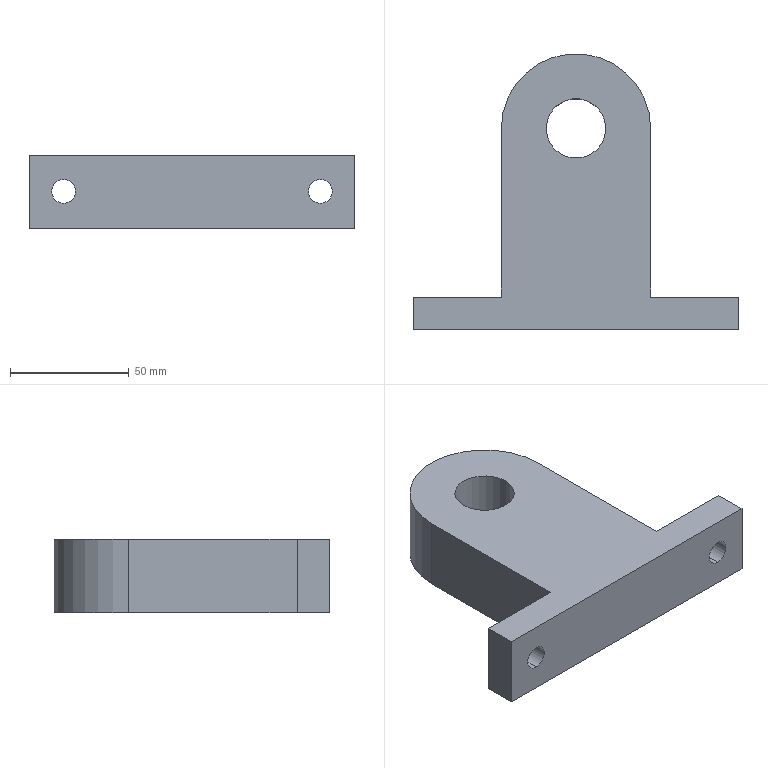Component | SolidWorks | BearingHousing-1 | 1 solid | 16 faces | box 137.01 x 116.01 x 31 mm | volume 226897 mm3 | plane 9 | cylinder 7 | commonest cylinder face diameters 10 x4 25 x2 62.794 x1
build123d program:
from build123d import *

# Parameters (mm, degrees)
SKETCH1_R           = 31.397
SKETCH1_R_2         = 12.5
BOSS_EXTRUDE1_DEPTH = 31
SKETCH2_R           = 5
CUT_EXTRUDE1_DEPTH  = 31


with BuildPart() as part:
    # Sketch1 → Boss-Extrude1 (new body)
    # profile 1 of 2: a face of its own
    with BuildSketch(Plane.XY):
        Circle(SKETCH1_R)
        with Locations(Location((0, 0, 0), (0, 0, 180))):
            Circle(SKETCH1_R_2, mode=Mode.SUBTRACT)
    # profile 2 of 2: a face of its own
    with BuildSketch(Plane.XY):
        with BuildLine():
            ThreePointArc((31.397, 0), (0, -31.397), (-31.397, 0))
            Line((-31.397, 0), (-31.397, -70.889))
            Line((-31.397, -70.889), (-68.507, -70.889))
            Line((-68.507, -70.889), (-68.507, -84.609))
            Line((-68.507, -84.609), (68.507, -84.609))
            Line((68.507, -84.609), (68.507, -70.889))
            Line((68.507, -70.889), (31.397, -70.889))
            Line((31.397, -70.889), (31.397, 0))
        make_face()
    extrude(amount=BOSS_EXTRUDE1_DEPTH)

    # Sketch2 → Cut-Extrude1 (cut)
    with BuildSketch(Plane(origin=(0, -70.889, 0), x_dir=(1, 0, 0), z_dir=(0, 1, 0))):
        with Locations(Location((54, -15.251, 0), (0, 0, 270))):
            Circle(SKETCH2_R)
        with Locations(Location((-54, -15.251, 0), (0, 0, 270))):
            Circle(SKETCH2_R)
    extrude(amount=-CUT_EXTRUDE1_DEPTH, mode=Mode.SUBTRACT)


solid = part.part

# Placed as in the assembly
solid = solid.moved(Location((0, 0, -146), (-180, 0, 180)))
STEP:
#1=CARTESIAN_POINT('',(2.126,-3.331,-6.545));
#2=VERTEX_POINT('',#1);
#3=CARTESIAN_POINT('',(2.126,-3.331,-6.152));
#4=VERTEX_POINT('',#3);
#5=CARTESIAN_POINT('',(2.126,-3.331,-6.348));
#6=DIRECTION('',(0.,-1.,0.));
#7=DIRECTION('',(0.,0.,-1.));
#8=AXIS2_PLACEMENT_3D('',#5,#6,#7);
#9=CIRCLE('',#8,0.1969);
#10=EDGE_CURVE('',#2,#4,#9,.T.);
#11=ORIENTED_EDGE('',*,*,#10,.T.);
#12=CARTESIAN_POINT('',(2.126,-2.791,-6.152));
#13=VERTEX_POINT('',#12);
#14=CARTESIAN_POINT('',(2.126,-4.011,-6.152));
#15=DIRECTION('',(0.,1.,0.));
#16=VECTOR('',#15,39.37);
#17=LINE('',#14,#16);
#18=EDGE_CURVE('',#4,#13,#17,.T.);
#19=ORIENTED_EDGE('',*,*,#18,.T.);
#20=CARTESIAN_POINT('',(2.126,-2.791,-6.545));
#21=VERTEX_POINT('',#20);
#22=CARTESIAN_POINT('',(2.126,-2.791,-6.348));
#23=DIRECTION('',(0.,-1.,0.));
#24=DIRECTION('',(0.,0.,-1.));
#25=AXIS2_PLACEMENT_3D('',#22,#23,#24);
#26=CIRCLE('',#25,0.1969);
#27=EDGE_CURVE('',#21,#13,#26,.T.);
#28=ORIENTED_EDGE('',*,*,#27,.F.);
#29=CARTESIAN_POINT('',(2.126,-4.011,-6.545));
#30=DIRECTION('',(0.,1.,0.));
#31=VECTOR('',#30,39.37);
#32=LINE('',#29,#31);
#33=EDGE_CURVE('',#2,#21,#32,.T.);
#34=ORIENTED_EDGE('',*,*,#33,.F.);
#35=EDGE_LOOP('',(#11,#19,#28,#34));
#36=FACE_OUTER_BOUND('',#35,.T.);
#37=CARTESIAN_POINT('',(2.126,-4.011,-6.348));
#38=DIRECTION('',(0.,1.,0.));
#39=DIRECTION('',(0.,0.,-1.));
#40=AXIS2_PLACEMENT_3D('',#37,#38,#39);
#41=CYLINDRICAL_SURFACE('',#40,0.1969);
#42=ADVANCED_FACE('',(#36),#41,.F.);
#43=CARTESIAN_POINT('',(-2.126,-3.331,-6.152));
#44=VERTEX_POINT('',#43);
#45=CARTESIAN_POINT('',(-2.126,-3.331,-6.545));
#46=VERTEX_POINT('',#45);
#47=CARTESIAN_POINT('',(-2.126,-3.331,-6.348));
#48=DIRECTION('',(0.,1.,0.));
#49=DIRECTION('',(0.,0.,-1.));
#50=AXIS2_PLACEMENT_3D('',#47,#48,#49);
#51=CIRCLE('',#50,0.1969);
#52=EDGE_CURVE('',#44,#46,#51,.T.);
#53=ORIENTED_EDGE('',*,*,#52,.F.);
#54=CARTESIAN_POINT('',(-2.126,-2.791,-6.152));
#55=VERTEX_POINT('',#54);
#56=CARTESIAN_POINT('',(-2.126,-4.011,-6.152));
#57=DIRECTION('',(0.,1.,0.));
#58=VECTOR('',#57,39.37);
#59=LINE('',#56,#58);
#60=EDGE_CURVE('',#44,#55,#59,.T.);
#61=ORIENTED_EDGE('',*,*,#60,.T.);
#62=CARTESIAN_POINT('',(-2.126,-2.791,-6.545));
#63=VERTEX_POINT('',#62);
#64=CARTESIAN_POINT('',(-2.126,-2.791,-6.348));
#65=DIRECTION('',(0.,1.,0.));
#66=DIRECTION('',(0.,0.,-1.));
#67=AXIS2_PLACEMENT_3D('',#64,#65,#66);
#68=CIRCLE('',#67,0.1969);
#69=EDGE_CURVE('',#55,#63,#68,.T.);
#70=ORIENTED_EDGE('',*,*,#69,.T.);
#71=CARTESIAN_POINT('',(-2.126,-4.011,-6.545));
#72=DIRECTION('',(0.,1.,0.));
#73=VECTOR('',#72,39.37);
#74=LINE('',#71,#73);
#75=EDGE_CURVE('',#46,#63,#74,.T.);
#76=ORIENTED_EDGE('',*,*,#75,.F.);
#77=EDGE_LOOP('',(#53,#61,#70,#76));
#78=FACE_OUTER_BOUND('',#77,.T.);
#79=CARTESIAN_POINT('',(-2.126,-4.011,-6.348));
#80=DIRECTION('',(0.,1.,0.));
#81=DIRECTION('',(0.,0.,-1.));
#82=AXIS2_PLACEMENT_3D('',#79,#80,#81);
#83=CYLINDRICAL_SURFACE('',#82,0.1969);
#84=ADVANCED_FACE('',(#78),#83,.F.);
#85=CARTESIAN_POINT('',(0.4921,0.,-6.969));
#86=VERTEX_POINT('',#85);
#87=CARTESIAN_POINT('',(-0.4921,0.,-6.969));
#88=VERTEX_POINT('',#87);
#89=CARTESIAN_POINT('',(0.,0.,-6.969));
#90=DIRECTION('',(0.,0.,-1.));
#91=DIRECTION('',(-1.,0.,0.));
#92=AXIS2_PLACEMENT_3D('',#89,#90,#91);
#93=CIRCLE('',#92,0.4921);
#94=EDGE_CURVE('',#86,#88,#93,.T.);
#95=ORIENTED_EDGE('',*,*,#94,.T.);
#96=CARTESIAN_POINT('',(-0.4921,0.,-5.748));
#97=VERTEX_POINT('',#96);
#98=CARTESIAN_POINT('',(-0.4921,0.,-6.969));
#99=DIRECTION('',(0.,0.,1.));
#100=VECTOR('',#99,39.37);
#101=LINE('',#98,#100);
#102=EDGE_CURVE('',#88,#97,#101,.T.);
#103=ORIENTED_EDGE('',*,*,#102,.T.);
#104=CARTESIAN_POINT('',(0.4921,0.,-5.748));
#105=VERTEX_POINT('',#104);
#106=CARTESIAN_POINT('',(0.,0.,-5.748));
#107=DIRECTION('',(0.,0.,-1.));
#108=DIRECTION('',(-1.,0.,0.));
#109=AXIS2_PLACEMENT_3D('',#106,#107,#108);
#110=CIRCLE('',#109,0.4921);
#111=EDGE_CURVE('',#105,#97,#110,.T.);
#112=ORIENTED_EDGE('',*,*,#111,.F.);
#113=CARTESIAN_POINT('',(0.4921,0.,-6.969));
#114=DIRECTION('',(0.,0.,1.));
#115=VECTOR('',#114,39.37);
#116=LINE('',#113,#115);
#117=EDGE_CURVE('',#86,#105,#116,.T.);
#118=ORIENTED_EDGE('',*,*,#117,.F.);
#119=EDGE_LOOP('',(#95,#103,#112,#118));
#120=FACE_OUTER_BOUND('',#119,.T.);
#121=CARTESIAN_POINT('',(0.,0.,-6.969));
#122=DIRECTION('',(0.,0.,1.));
#123=DIRECTION('',(1.,0.,0.));
#124=AXIS2_PLACEMENT_3D('',#121,#122,#123);
#125=CYLINDRICAL_SURFACE('',#124,0.4921);
#126=ADVANCED_FACE('',(#120),#125,.F.);
#127=CARTESIAN_POINT('',(2.697,-3.331,-5.748));
#128=VERTEX_POINT('',#127);
#129=CARTESIAN_POINT('',(-2.697,-3.331,-5.748));
#130=VERTEX_POINT('',#129);
#131=CARTESIAN_POINT('',(0.,-3.331,-5.748));
#132=DIRECTION('',(-1.,0.,0.));
#133=VECTOR('',#132,39.37);
#134=LINE('',#131,#133);
#135=EDGE_CURVE('',#128,#130,#134,.T.);
#136=ORIENTED_EDGE('',*,*,#135,.T.);
#137=CARTESIAN_POINT('',(-2.697,-3.331,-6.969));
#138=VERTEX_POINT('',#137);
#139=CARTESIAN_POINT('',(-2.697,-3.331,-6.969));
#140=DIRECTION('',(0.,0.,1.));
#141=VECTOR('',#140,39.37);
#142=LINE('',#139,#141);
#143=EDGE_CURVE('',#138,#130,#142,.T.);
#144=ORIENTED_EDGE('',*,*,#143,.F.);
#145=CARTESIAN_POINT('',(2.697,-3.331,-6.969));
#146=VERTEX_POINT('',#145);
#147=CARTESIAN_POINT('',(0.,-3.331,-6.969));
#148=DIRECTION('',(-1.,0.,0.));
#149=VECTOR('',#148,39.37);
#150=LINE('',#147,#149);
#151=EDGE_CURVE('',#146,#138,#150,.T.);
#152=ORIENTED_EDGE('',*,*,#151,.F.);
#153=CARTESIAN_POINT('',(2.697,-3.331,-6.969));
#154=DIRECTION('',(0.,0.,1.));
#155=VECTOR('',#154,39.37);
#156=LINE('',#153,#155);
#157=EDGE_CURVE('',#146,#128,#156,.T.);
#158=ORIENTED_EDGE('',*,*,#157,.T.);
#159=EDGE_LOOP('',(#136,#144,#152,#158));
#160=FACE_OUTER_BOUND('',#159,.T.);
#161=ORIENTED_EDGE('',*,*,#10,.F.);
#162=CARTESIAN_POINT('',(2.126,-3.331,-6.348));
#163=DIRECTION('',(0.,-1.,0.));
#164=DIRECTION('',(0.,0.,-1.));
#165=AXIS2_PLACEMENT_3D('',#162,#163,#164);
#166=CIRCLE('',#165,0.1969);
#167=EDGE_CURVE('',#4,#2,#166,.T.);
#168=ORIENTED_EDGE('',*,*,#167,.F.);
#169=EDGE_LOOP('',(#161,#168));
#170=FACE_BOUND('',#169,.T.);
#171=CARTESIAN_POINT('',(-2.126,-3.331,-6.348));
#172=DIRECTION('',(0.,1.,0.));
#173=DIRECTION('',(0.,0.,-1.));
#174=AXIS2_PLACEMENT_3D('',#171,#172,#173);
#175=CIRCLE('',#174,0.1969);
#176=EDGE_CURVE('',#46,#44,#175,.T.);
#177=ORIENTED_EDGE('',*,*,#176,.T.);
#178=ORIENTED_EDGE('',*,*,#52,.T.);
#179=EDGE_LOOP('',(#177,#178));
#180=FACE_BOUND('',#179,.T.);
#181=CARTESIAN_POINT('',(0.,-3.331,-6.969));
#182=DIRECTION('',(0.,1.,0.));
#183=DIRECTION('',(0.,0.,-1.));
#184=AXIS2_PLACEMENT_3D('',#181,#182,#183);
#185=PLANE('',#184);
#186=ADVANCED_FACE('',(#160,#170,#180),#185,.F.);
#187=CARTESIAN_POINT('',(-1.236,0.,-5.748));
#188=VERTEX_POINT('',#187);
#189=CARTESIAN_POINT('',(1.236,0.,-5.748));
#190=VERTEX_POINT('',#189);
#191=CARTESIAN_POINT('',(0.,0.,-5.748));
#192=DIRECTION('',(0.,0.,-1.));
#193=DIRECTION('',(-1.,0.,0.));
#194=AXIS2_PLACEMENT_3D('',#191,#192,#193);
#195=CIRCLE('',#194,1.236);
#196=EDGE_CURVE('',#188,#190,#195,.T.);
#197=ORIENTED_EDGE('',*,*,#196,.T.);
#198=CARTESIAN_POINT('',(1.236,0.,-6.969));
#199=VERTEX_POINT('',#198);
#200=CARTESIAN_POINT('',(1.236,0.,-6.969));
#201=DIRECTION('',(0.,0.,1.));
#202=VECTOR('',#201,39.37);
#203=LINE('',#200,#202);
#204=EDGE_CURVE('',#199,#190,#203,.T.);
#205=ORIENTED_EDGE('',*,*,#204,.F.);
#206=CARTESIAN_POINT('',(-1.236,0.,-6.969));
#207=VERTEX_POINT('',#206);
#208=CARTESIAN_POINT('',(0.,0.,-6.969));
#209=DIRECTION('',(0.,0.,-1.));
#210=DIRECTION('',(-1.,0.,0.));
#211=AXIS2_PLACEMENT_3D('',#208,#209,#210);
#212=CIRCLE('',#211,1.236);
#213=EDGE_CURVE('',#207,#199,#212,.T.);
#214=ORIENTED_EDGE('',*,*,#213,.F.);
#215=CARTESIAN_POINT('',(-1.236,0.,-6.969));
#216=DIRECTION('',(0.,0.,1.));
#217=VECTOR('',#216,39.37);
#218=LINE('',#215,#217);
#219=EDGE_CURVE('',#207,#188,#218,.T.);
#220=ORIENTED_EDGE('',*,*,#219,.T.);
#221=EDGE_LOOP('',(#197,#205,#214,#220));
#222=FACE_OUTER_BOUND('',#221,.T.);
#223=CARTESIAN_POINT('',(0.,0.,-6.969));
#224=DIRECTION('',(0.,0.,1.));
#225=DIRECTION('',(1.,0.,0.));
#226=AXIS2_PLACEMENT_3D('',#223,#224,#225);
#227=CYLINDRICAL_SURFACE('',#226,1.236);
#228=ADVANCED_FACE('',(#222),#227,.T.);
#229=CARTESIAN_POINT('',(1.236,-2.791,-5.748));
#230=VERTEX_POINT('',#229);
#231=CARTESIAN_POINT('',(1.236,0.,-5.748));
#232=DIRECTION('',(0.,-1.,0.));
#233=VECTOR('',#232,39.37);
#234=LINE('',#231,#233);
#235=EDGE_CURVE('',#190,#230,#234,.T.);
#236=ORIENTED_EDGE('',*,*,#235,.T.);
#237=CARTESIAN_POINT('',(1.236,-2.791,-6.969));
#238=VERTEX_POINT('',#237);
#239=CARTESIAN_POINT('',(1.236,-2.791,-6.969));
#240=DIRECTION('',(0.,0.,1.));
#241=VECTOR('',#240,39.37);
#242=LINE('',#239,#241);
#243=EDGE_CURVE('',#238,#230,#242,.T.);
#244=ORIENTED_EDGE('',*,*,#243,.F.);
#245=CARTESIAN_POINT('',(1.236,0.,-6.969));
#246=DIRECTION('',(0.,-1.,0.));
#247=VECTOR('',#246,39.37);
#248=LINE('',#245,#247);
#249=EDGE_CURVE('',#199,#238,#248,.T.);
#250=ORIENTED_EDGE('',*,*,#249,.F.);
#251=ORIENTED_EDGE('',*,*,#204,.T.);
#252=EDGE_LOOP('',(#236,#244,#250,#251));
#253=FACE_OUTER_BOUND('',#252,.T.);
#254=CARTESIAN_POINT('',(1.236,0.,-6.969));
#255=DIRECTION('',(-1.,0.,0.));
#256=DIRECTION('',(0.,0.,1.));
#257=AXIS2_PLACEMENT_3D('',#254,#255,#256);
#258=PLANE('',#257);
#259=ADVANCED_FACE('',(#253),#258,.F.);
#260=ORIENTED_EDGE('',*,*,#27,.T.);
#261=CARTESIAN_POINT('',(2.126,-2.791,-6.348));
#262=DIRECTION('',(0.,-1.,0.));
#263=DIRECTION('',(0.,0.,-1.));
#264=AXIS2_PLACEMENT_3D('',#261,#262,#263);
#265=CIRCLE('',#264,0.1969);
#266=EDGE_CURVE('',#13,#21,#265,.T.);
#267=ORIENTED_EDGE('',*,*,#266,.T.);
#268=EDGE_LOOP('',(#260,#267));
#269=FACE_BOUND('',#268,.T.);
#270=CARTESIAN_POINT('',(2.697,-2.791,-5.748));
#271=VERTEX_POINT('',#270);
#272=CARTESIAN_POINT('',(0.,-2.791,-5.748));
#273=DIRECTION('',(1.,0.,0.));
#274=VECTOR('',#273,39.37);
#275=LINE('',#272,#274);
#276=EDGE_CURVE('',#230,#271,#275,.T.);
#277=ORIENTED_EDGE('',*,*,#276,.T.);
#278=CARTESIAN_POINT('',(2.697,-2.791,-6.969));
#279=VERTEX_POINT('',#278);
#280=CARTESIAN_POINT('',(2.697,-2.791,-6.969));
#281=DIRECTION('',(0.,0.,1.));
#282=VECTOR('',#281,39.37);
#283=LINE('',#280,#282);
#284=EDGE_CURVE('',#279,#271,#283,.T.);
#285=ORIENTED_EDGE('',*,*,#284,.F.);
#286=CARTESIAN_POINT('',(0.,-2.791,-6.969));
#287=DIRECTION('',(1.,0.,0.));
#288=VECTOR('',#287,39.37);
#289=LINE('',#286,#288);
#290=EDGE_CURVE('',#238,#279,#289,.T.);
#291=ORIENTED_EDGE('',*,*,#290,.F.);
#292=ORIENTED_EDGE('',*,*,#243,.T.);
#293=EDGE_LOOP('',(#277,#285,#291,#292));
#294=FACE_OUTER_BOUND('',#293,.T.);
#295=CARTESIAN_POINT('',(0.,-2.791,-6.969));
#296=DIRECTION('',(0.,-1.,0.));
#297=DIRECTION('',(0.,0.,1.));
#298=AXIS2_PLACEMENT_3D('',#295,#296,#297);
#299=PLANE('',#298);
#300=ADVANCED_FACE('',(#269,#294),#299,.F.);
#301=CARTESIAN_POINT('',(2.697,0.,-5.748));
#302=DIRECTION('',(0.,-1.,0.));
#303=VECTOR('',#302,39.37);
#304=LINE('',#301,#303);
#305=EDGE_CURVE('',#271,#128,#304,.T.);
#306=ORIENTED_EDGE('',*,*,#305,.T.);
#307=ORIENTED_EDGE('',*,*,#157,.F.);
#308=CARTESIAN_POINT('',(2.697,0.,-6.969));
#309=DIRECTION('',(0.,-1.,0.));
#310=VECTOR('',#309,39.37);
#311=LINE('',#308,#310);
#312=EDGE_CURVE('',#279,#146,#311,.T.);
#313=ORIENTED_EDGE('',*,*,#312,.F.);
#314=ORIENTED_EDGE('',*,*,#284,.T.);
#315=EDGE_LOOP('',(#306,#307,#313,#314));
#316=FACE_OUTER_BOUND('',#315,.T.);
#317=CARTESIAN_POINT('',(2.697,0.,-6.969));
#318=DIRECTION('',(-1.,0.,0.));
#319=DIRECTION('',(0.,0.,1.));
#320=AXIS2_PLACEMENT_3D('',#317,#318,#319);
#321=PLANE('',#320);
#322=ADVANCED_FACE('',(#316),#321,.F.);
#323=CARTESIAN_POINT('',(-2.697,-2.791,-5.748));
#324=VERTEX_POINT('',#323);
#325=CARTESIAN_POINT('',(-2.697,0.,-5.748));
#326=DIRECTION('',(0.,-1.,0.));
#327=VECTOR('',#326,39.37);
#328=LINE('',#325,#327);
#329=EDGE_CURVE('',#324,#130,#328,.T.);
#330=ORIENTED_EDGE('',*,*,#329,.F.);
#331=CARTESIAN_POINT('',(-2.697,-2.791,-6.969));
#332=VERTEX_POINT('',#331);
#333=CARTESIAN_POINT('',(-2.697,-2.791,-6.969));
#334=DIRECTION('',(0.,0.,1.));
#335=VECTOR('',#334,39.37);
#336=LINE('',#333,#335);
#337=EDGE_CURVE('',#332,#324,#336,.T.);
#338=ORIENTED_EDGE('',*,*,#337,.F.);
#339=CARTESIAN_POINT('',(-2.697,0.,-6.969));
#340=DIRECTION('',(0.,-1.,0.));
#341=VECTOR('',#340,39.37);
#342=LINE('',#339,#341);
#343=EDGE_CURVE('',#332,#138,#342,.T.);
#344=ORIENTED_EDGE('',*,*,#343,.T.);
#345=ORIENTED_EDGE('',*,*,#143,.T.);
#346=EDGE_LOOP('',(#330,#338,#344,#345));
#347=FACE_OUTER_BOUND('',#346,.T.);
#348=CARTESIAN_POINT('',(-2.697,0.,-6.969));
#349=DIRECTION('',(-1.,0.,0.));
#350=DIRECTION('',(0.,0.,1.));
#351=AXIS2_PLACEMENT_3D('',#348,#349,#350);
#352=PLANE('',#351);
#353=ADVANCED_FACE('',(#347),#352,.T.);
#354=CARTESIAN_POINT('',(-2.126,-2.791,-6.348));
#355=DIRECTION('',(0.,1.,0.));
#356=DIRECTION('',(0.,0.,-1.));
#357=AXIS2_PLACEMENT_3D('',#354,#355,#356);
#358=CIRCLE('',#357,0.1969);
#359=EDGE_CURVE('',#63,#55,#358,.T.);
#360=ORIENTED_EDGE('',*,*,#359,.F.);
#361=ORIENTED_EDGE('',*,*,#69,.F.);
#362=EDGE_LOOP('',(#360,#361));
#363=FACE_BOUND('',#362,.T.);
#364=CARTESIAN_POINT('',(-1.236,-2.791,-5.748));
#365=VERTEX_POINT('',#364);
#366=CARTESIAN_POINT('',(0.,-2.791,-5.748));
#367=DIRECTION('',(-1.,0.,0.));
#368=VECTOR('',#367,39.37);
#369=LINE('',#366,#368);
#370=EDGE_CURVE('',#365,#324,#369,.T.);
#371=ORIENTED_EDGE('',*,*,#370,.F.);
#372=CARTESIAN_POINT('',(-1.236,-2.791,-6.969));
#373=VERTEX_POINT('',#372);
#374=CARTESIAN_POINT('',(-1.236,-2.791,-6.969));
#375=DIRECTION('',(0.,0.,1.));
#376=VECTOR('',#375,39.37);
#377=LINE('',#374,#376);
#378=EDGE_CURVE('',#373,#365,#377,.T.);
#379=ORIENTED_EDGE('',*,*,#378,.F.);
#380=CARTESIAN_POINT('',(0.,-2.791,-6.969));
#381=DIRECTION('',(-1.,0.,0.));
#382=VECTOR('',#381,39.37);
#383=LINE('',#380,#382);
#384=EDGE_CURVE('',#373,#332,#383,.T.);
#385=ORIENTED_EDGE('',*,*,#384,.T.);
#386=ORIENTED_EDGE('',*,*,#337,.T.);
#387=EDGE_LOOP('',(#371,#379,#385,#386));
#388=FACE_OUTER_BOUND('',#387,.T.);
#389=CARTESIAN_POINT('',(0.,-2.791,-6.969));
#390=DIRECTION('',(0.,1.,0.));
#391=DIRECTION('',(0.,0.,-1.));
#392=AXIS2_PLACEMENT_3D('',#389,#390,#391);
#393=PLANE('',#392);
#394=ADVANCED_FACE('',(#363,#388),#393,.T.);
#395=ORIENTED_EDGE('',*,*,#102,.F.);
#396=CARTESIAN_POINT('',(0.,0.,-6.969));
#397=DIRECTION('',(0.,0.,-1.));
#398=DIRECTION('',(-1.,0.,0.));
#399=AXIS2_PLACEMENT_3D('',#396,#397,#398);
#400=CIRCLE('',#399,0.4921);
#401=EDGE_CURVE('',#88,#86,#400,.T.);
#402=ORIENTED_EDGE('',*,*,#401,.T.);
#403=ORIENTED_EDGE('',*,*,#117,.T.);
#404=CARTESIAN_POINT('',(0.,0.,-5.748));
#405=DIRECTION('',(0.,0.,-1.));
#406=DIRECTION('',(-1.,0.,0.));
#407=AXIS2_PLACEMENT_3D('',#404,#405,#406);
#408=CIRCLE('',#407,0.4921);
#409=EDGE_CURVE('',#97,#105,#408,.T.);
#410=ORIENTED_EDGE('',*,*,#409,.F.);
#411=EDGE_LOOP('',(#395,#402,#403,#410));
#412=FACE_OUTER_BOUND('',#411,.T.);
#413=CARTESIAN_POINT('',(0.,0.,-6.969));
#414=DIRECTION('',(0.,0.,1.));
#415=DIRECTION('',(1.,0.,0.));
#416=AXIS2_PLACEMENT_3D('',#413,#414,#415);
#417=CYLINDRICAL_SURFACE('',#416,0.4921);
#418=ADVANCED_FACE('',(#412),#417,.F.);
#419=CARTESIAN_POINT('',(-1.236,0.,-5.748));
#420=DIRECTION('',(0.,-1.,0.));
#421=VECTOR('',#420,39.37);
#422=LINE('',#419,#421);
#423=EDGE_CURVE('',#188,#365,#422,.T.);
#424=ORIENTED_EDGE('',*,*,#423,.F.);
#425=ORIENTED_EDGE('',*,*,#219,.F.);
#426=CARTESIAN_POINT('',(-1.236,0.,-6.969));
#427=DIRECTION('',(0.,-1.,0.));
#428=VECTOR('',#427,39.37);
#429=LINE('',#426,#428);
#430=EDGE_CURVE('',#207,#373,#429,.T.);
#431=ORIENTED_EDGE('',*,*,#430,.T.);
#432=ORIENTED_EDGE('',*,*,#378,.T.);
#433=EDGE_LOOP('',(#424,#425,#431,#432));
#434=FACE_OUTER_BOUND('',#433,.T.);
#435=CARTESIAN_POINT('',(-1.236,0.,-6.969));
#436=DIRECTION('',(-1.,0.,0.));
#437=DIRECTION('',(0.,0.,1.));
#438=AXIS2_PLACEMENT_3D('',#435,#436,#437);
#439=PLANE('',#438);
#440=ADVANCED_FACE('',(#434),#439,.T.);
#441=ORIENTED_EDGE('',*,*,#94,.F.);
#442=ORIENTED_EDGE('',*,*,#401,.F.);
#443=EDGE_LOOP('',(#441,#442));
#444=FACE_BOUND('',#443,.T.);
#445=ORIENTED_EDGE('',*,*,#213,.T.);
#446=ORIENTED_EDGE('',*,*,#249,.T.);
#447=ORIENTED_EDGE('',*,*,#290,.T.);
#448=ORIENTED_EDGE('',*,*,#312,.T.);
#449=ORIENTED_EDGE('',*,*,#151,.T.);
#450=ORIENTED_EDGE('',*,*,#343,.F.);
#451=ORIENTED_EDGE('',*,*,#384,.F.);
#452=ORIENTED_EDGE('',*,*,#430,.F.);
#453=EDGE_LOOP('',(#445,#446,#447,#448,#449,#450,#451,#452));
#454=FACE_OUTER_BOUND('',#453,.T.);
#455=CARTESIAN_POINT('',(0.,0.,-6.969));
#456=DIRECTION('',(0.,0.,-1.));
#457=DIRECTION('',(-1.,0.,0.));
#458=AXIS2_PLACEMENT_3D('',#455,#456,#457);
#459=PLANE('',#458);
#460=ADVANCED_FACE('',(#444,#454),#459,.T.);
#461=ORIENTED_EDGE('',*,*,#111,.T.);
#462=ORIENTED_EDGE('',*,*,#409,.T.);
#463=EDGE_LOOP('',(#461,#462));
#464=FACE_BOUND('',#463,.T.);
#465=ORIENTED_EDGE('',*,*,#196,.F.);
#466=ORIENTED_EDGE('',*,*,#423,.T.);
#467=ORIENTED_EDGE('',*,*,#370,.T.);
#468=ORIENTED_EDGE('',*,*,#329,.T.);
#469=ORIENTED_EDGE('',*,*,#135,.F.);
#470=ORIENTED_EDGE('',*,*,#305,.F.);
#471=ORIENTED_EDGE('',*,*,#276,.F.);
#472=ORIENTED_EDGE('',*,*,#235,.F.);
#473=EDGE_LOOP('',(#465,#466,#467,#468,#469,#470,#471,#472));
#474=FACE_OUTER_BOUND('',#473,.T.);
#475=CARTESIAN_POINT('',(0.,0.,-5.748));
#476=DIRECTION('',(0.,0.,-1.));
#477=DIRECTION('',(-1.,0.,0.));
#478=AXIS2_PLACEMENT_3D('',#475,#476,#477);
#479=PLANE('',#478);
#480=ADVANCED_FACE('',(#464,#474),#479,.F.);
#481=ORIENTED_EDGE('',*,*,#60,.F.);
#482=ORIENTED_EDGE('',*,*,#176,.F.);
#483=ORIENTED_EDGE('',*,*,#75,.T.);
#484=ORIENTED_EDGE('',*,*,#359,.T.);
#485=EDGE_LOOP('',(#481,#482,#483,#484));
#486=FACE_OUTER_BOUND('',#485,.T.);
#487=CARTESIAN_POINT('',(-2.126,-4.011,-6.348));
#488=DIRECTION('',(0.,1.,0.));
#489=DIRECTION('',(0.,0.,-1.));
#490=AXIS2_PLACEMENT_3D('',#487,#488,#489);
#491=CYLINDRICAL_SURFACE('',#490,0.1969);
#492=ADVANCED_FACE('',(#486),#491,.F.);
#493=ORIENTED_EDGE('',*,*,#18,.F.);
#494=ORIENTED_EDGE('',*,*,#167,.T.);
#495=ORIENTED_EDGE('',*,*,#33,.T.);
#496=ORIENTED_EDGE('',*,*,#266,.F.);
#497=EDGE_LOOP('',(#493,#494,#495,#496));
#498=FACE_OUTER_BOUND('',#497,.T.);
#499=CARTESIAN_POINT('',(2.126,-4.011,-6.348));
#500=DIRECTION('',(0.,1.,0.));
#501=DIRECTION('',(0.,0.,-1.));
#502=AXIS2_PLACEMENT_3D('',#499,#500,#501);
#503=CYLINDRICAL_SURFACE('',#502,0.1969);
#504=ADVANCED_FACE('',(#498),#503,.F.);
#505=CLOSED_SHELL('',(#42,#84,#126,#186,#228,#259,#300,#322,#353,#394,#418,#440,#460,#480,#492,#504));
#506=MANIFOLD_SOLID_BREP('',#505);
#507=CARTESIAN_POINT('',(0.,0.,0.));
#508=DIRECTION('',(0.,0.,1.));
#509=DIRECTION('',(1.,0.,0.));
#510=AXIS2_PLACEMENT_3D('',#507,#508,#509);
#511=(LENGTH_UNIT()NAMED_UNIT(*)SI_UNIT($,.METRE.));
#512=LENGTH_MEASURE_WITH_UNIT(LENGTH_MEASURE(0.0254),#511);
#513=DIMENSIONAL_EXPONENTS(1.,0.,0.,0.,0.,0.,0.);
#514=(CONVERSION_BASED_UNIT('',#512)LENGTH_UNIT()NAMED_UNIT(#513));
#515=UNCERTAINTY_MEASURE_WITH_UNIT(LENGTH_MEASURE(0.00001),#514,'','');
#516=(NAMED_UNIT(*)PLANE_ANGLE_UNIT()SI_UNIT($,.RADIAN.));
#517=(NAMED_UNIT(*)SI_UNIT($,.STERADIAN.)SOLID_ANGLE_UNIT());
#518=(GEOMETRIC_REPRESENTATION_CONTEXT(3)GLOBAL_UNCERTAINTY_ASSIGNED_CONTEXT((#515))GLOBAL_UNIT_ASSIGNED_CONTEXT((#514,#516,#517))REPRESENTATION_CONTEXT('',''));
#519=ADVANCED_BREP_SHAPE_REPRESENTATION('',(#506,#510),#518);
#520=COLOUR_RGB('',0.7922,0.8196,0.9333);
#521=FILL_AREA_STYLE_COLOUR('',#520);
#522=FILL_AREA_STYLE('',(#521));
#523=SURFACE_STYLE_FILL_AREA(#522);
#524=SURFACE_SIDE_STYLE('',(#523));
#525=SURFACE_STYLE_USAGE(.BOTH.,#524);
#526=PRESENTATION_STYLE_ASSIGNMENT((#525));
#527=STYLED_ITEM('',(#526),#506);
#528=(LENGTH_UNIT()NAMED_UNIT(*)SI_UNIT($,.METRE.));
#529=LENGTH_MEASURE_WITH_UNIT(LENGTH_MEASURE(0.0254),#528);
#530=DIMENSIONAL_EXPONENTS(1.,0.,0.,0.,0.,0.,0.);
#531=(CONVERSION_BASED_UNIT('',#529)LENGTH_UNIT()NAMED_UNIT(#530));
#532=UNCERTAINTY_MEASURE_WITH_UNIT(LENGTH_MEASURE(0.00001),#531,'','');
#533=(NAMED_UNIT(*)PLANE_ANGLE_UNIT()SI_UNIT($,.RADIAN.));
#534=(NAMED_UNIT(*)SI_UNIT($,.STERADIAN.)SOLID_ANGLE_UNIT());
#535=(GEOMETRIC_REPRESENTATION_CONTEXT(3)GLOBAL_UNCERTAINTY_ASSIGNED_CONTEXT((#532))GLOBAL_UNIT_ASSIGNED_CONTEXT((#531,#533,#534))REPRESENTATION_CONTEXT('',''));
#536=MECHANICAL_DESIGN_GEOMETRIC_PRESENTATION_REPRESENTATION('',(#527),#535);
#537=PRESENTATION_LAYER_ASSIGNMENT('','',(#527));